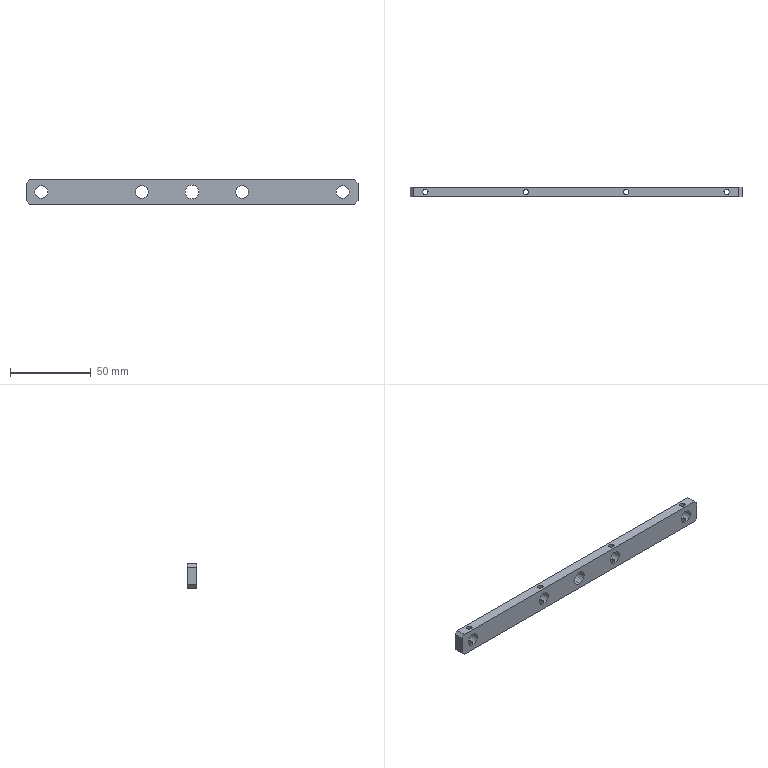Component | SolidWorks | 04LowerMaterialReceivingSwingAngleAssembly(3920)-1_H2020022-0448-1(3920)-3 | 1 solid | 36 faces | box 205 x 6 x 15 mm | volume 16610 mm3 | cylinder 26 | plane 10 | commonest cylinder face diameters 3.3 x16 8 x8 8.5 x2 | material 45#Steel
build123d program:
from build123d import *

# Parameters (mm, degrees)
SKETCH1_W           = 205
SKETCH1_H           = 15
BOSS_EXTRUDE1_DEPTH = 6
SKETCH2_R           = 4
CUT_EXTRUDE1_DEPTH  = 206.636
M4_TAPPED_HOLE1_D   = 3.3
LPATTERN2_COUNT     = 4
LPATTERN2_PITCH     = 62
CHAMFER3_SIZE       = 2
SKETCH8_R           = 4.25
CUT_EXTRUDE2_DEPTH  = 206.636


with BuildPart() as part:
    # Sketch1 → Boss-Extrude1 (new body)
    with BuildSketch(Plane(origin=(0, 0, 0), x_dir=(1, 0, 0), z_dir=(0, 1, 0))):
        with Locations((102.5, -7.5)):
            Rectangle(SKETCH1_W, SKETCH1_H)
    extrude(amount=BOSS_EXTRUDE1_DEPTH)

    # Sketch2 → Cut-Extrude1 (cut, through all)
    with BuildSketch(Plane(origin=(0, 6, 0), x_dir=(1, 0, 0), z_dir=(0, 1, 0))):
        with Locations(Location((9.5, -7.5, 0), (0, 0, 270))):
            Circle(SKETCH2_R)
    cut_extrude1 = extrude(amount=-CUT_EXTRUDE1_DEPTH, mode=Mode.SUBTRACT)

    # M4 Tapped Hole1 (through all)
    with Locations(Plane.XY.offset(15)):
        with Locations((9.5, 3)):
            m4_tapped_hole1 = Hole(M4_TAPPED_HOLE1_D / 2)

    # LPattern2: Cut-Extrude1, M4 Tapped Hole1 ×4
    with Locations(*[(i * LPATTERN2_PITCH, 0, 0) for i in range(1, LPATTERN2_COUNT)]):
        add(cut_extrude1, mode=Mode.SUBTRACT)
        add(m4_tapped_hole1, mode=Mode.SUBTRACT)

    # Chamfer3
    chamfer3_edges = [part.edges().sort_by_distance(p)[0] for p in [
        (0, 3, 0),
        (205, 3, 0),
        (205, 3, 15),
        (0, 3, 15),
    ]]
    chamfer(chamfer3_edges, length=CHAMFER3_SIZE)

    # Sketch8 → Cut-Extrude2 (cut, through all)
    with BuildSketch(Plane(origin=(0, 6, 0), x_dir=(1, 0, 0), z_dir=(0, 1, 0))):
        with Locations(Location((102.5, -7.5, 0), (0, 0, 270))):
            Circle(SKETCH8_R)
    extrude(amount=-CUT_EXTRUDE2_DEPTH, mode=Mode.SUBTRACT)


solid = part.part

# Placed as in the assembly
solid = solid.moved(Location((-133.464, 184.813, 272.697), (0, 0, 0)))